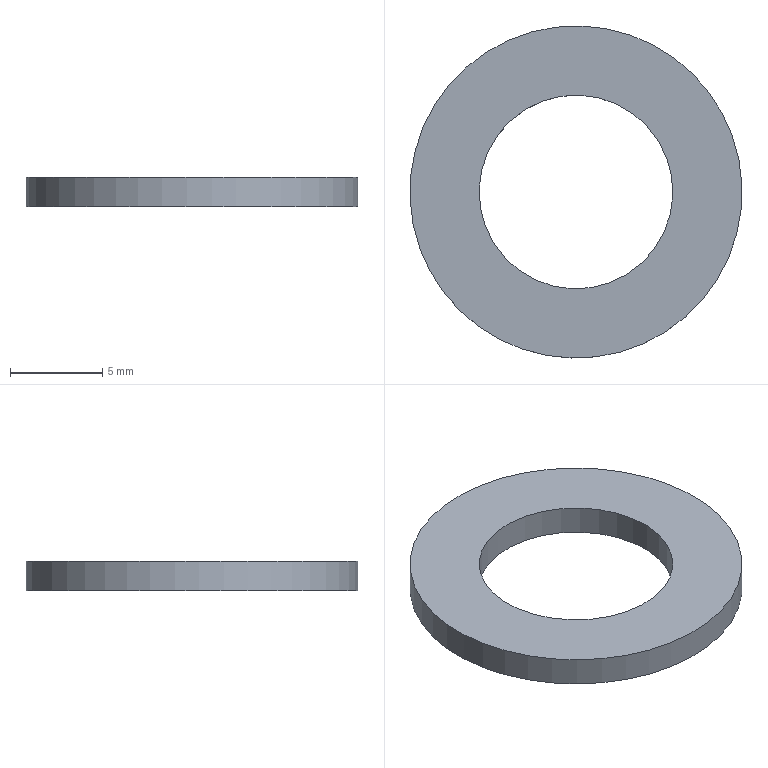Component | NX | CA6140-ZHUZHOU-DIANQUAN | 1 solid | 4 faces | box 18 x 18 x 1.6 mm | volume 269 mm3 | cylinder 2 | plane 2 | commonest cylinder face diameters 18 x1 10.5 x1
STEP:
#1=CARTESIAN_POINT('',(0.,0.,0.));
#2=DIRECTION('',(0.,0.,1.));
#3=DIRECTION('',(1.,0.,0.));
#4=AXIS2_PLACEMENT_3D('',#1,#2,#3);
#5=CARTESIAN_POINT('',(-61.859,-63.85,110.4));
#6=VERTEX_POINT('',#5);
#7=CARTESIAN_POINT('',(-56.569,-56.569,110.4));
#8=DIRECTION('',(0.,0.,1.));
#9=DIRECTION('',(-0.5878,-0.809,0.));
#10=AXIS2_PLACEMENT_3D('',#7,#8,#9);
#11=CIRCLE('',#10,9.);
#12=CARTESIAN_POINT('',(-56.569,-56.569,110.4));
#13=DIRECTION('',(0.,0.,1.));
#14=DIRECTION('',(0.5878,0.809,0.));
#15=AXIS2_PLACEMENT_3D('',#12,#13,#14);
#16=CYLINDRICAL_SURFACE('',#15,9.);
#17=CARTESIAN_POINT('',(3.142,0.));
#18=DIRECTION('',(1.,0.));
#19=VECTOR('',#18,1.);
#20=LINE('',#17,#19);
#21=(GEOMETRIC_REPRESENTATION_CONTEXT(2)PARAMETRIC_REPRESENTATION_CONTEXT()REPRESENTATION_CONTEXT('',''));
#22=DEFINITIONAL_REPRESENTATION('',(#20),#21);
#23=PCURVE('',#16,#22);
#24=CARTESIAN_POINT('',(-56.569,-56.569,110.4));
#25=DIRECTION('',(0.,0.,1.));
#26=DIRECTION('',(0.5878,0.809,0.));
#27=AXIS2_PLACEMENT_3D('',#24,#25,#26);
#28=PLANE('',#27);
#29=CARTESIAN_POINT('',(0.,0.));
#30=DIRECTION('',(-1.,0.));
#31=AXIS2_PLACEMENT_2D('',#29,#30);
#32=CIRCLE('',#31,9.);
#33=(GEOMETRIC_REPRESENTATION_CONTEXT(2)PARAMETRIC_REPRESENTATION_CONTEXT()REPRESENTATION_CONTEXT('',''));
#34=DEFINITIONAL_REPRESENTATION('',(#32),#33);
#35=PCURVE('',#28,#34);
#36=SURFACE_CURVE('',#11,(#23,#35),.PCURVE_S1.);
#37=EDGE_CURVE('',#6,#6,#36,.T.);
#38=ORIENTED_EDGE('',*,*,#37,.T.);
#39=CARTESIAN_POINT('',(-61.859,-63.85,112.));
#40=VERTEX_POINT('',#39);
#41=CARTESIAN_POINT('',(-61.859,-63.85,110.4));
#42=CARTESIAN_POINT('',(-61.859,-63.85,112.));
#43=B_SPLINE_CURVE_WITH_KNOTS('',1,(#41,#42),.UNSPECIFIED.,.F.,.F.,(2,2),(0.,1.6),.PIECEWISE_BEZIER_KNOTS.);
#44=CARTESIAN_POINT('',(9.425,0.));
#45=DIRECTION('',(0.,1.));
#46=VECTOR('',#45,1.);
#47=LINE('',#44,#46);
#48=(GEOMETRIC_REPRESENTATION_CONTEXT(2)PARAMETRIC_REPRESENTATION_CONTEXT()REPRESENTATION_CONTEXT('',''));
#49=DEFINITIONAL_REPRESENTATION('',(#47),#48);
#50=PCURVE('',#16,#49);
#51=CARTESIAN_POINT('',(3.142,0.));
#52=DIRECTION('',(0.,1.));
#53=VECTOR('',#52,1.);
#54=LINE('',#51,#53);
#55=(GEOMETRIC_REPRESENTATION_CONTEXT(2)PARAMETRIC_REPRESENTATION_CONTEXT()REPRESENTATION_CONTEXT('',''));
#56=DEFINITIONAL_REPRESENTATION('',(#54),#55);
#57=PCURVE('',#16,#56);
#58=SEAM_CURVE('',#43,(#50,#57),.PCURVE_S1.);
#59=EDGE_CURVE('',#6,#40,#58,.T.);
#60=ORIENTED_EDGE('',*,*,#59,.T.);
#61=CARTESIAN_POINT('',(-56.569,-56.569,112.));
#62=DIRECTION('',(0.,0.,1.));
#63=DIRECTION('',(-0.5878,-0.809,0.));
#64=AXIS2_PLACEMENT_3D('',#61,#62,#63);
#65=CIRCLE('',#64,9.);
#66=CARTESIAN_POINT('',(3.142,1.6));
#67=DIRECTION('',(1.,0.));
#68=VECTOR('',#67,1.);
#69=LINE('',#66,#68);
#70=(GEOMETRIC_REPRESENTATION_CONTEXT(2)PARAMETRIC_REPRESENTATION_CONTEXT()REPRESENTATION_CONTEXT('',''));
#71=DEFINITIONAL_REPRESENTATION('',(#69),#70);
#72=PCURVE('',#16,#71);
#73=CARTESIAN_POINT('',(-56.569,-56.569,112.));
#74=DIRECTION('',(0.,0.,1.));
#75=DIRECTION('',(0.5878,0.809,0.));
#76=AXIS2_PLACEMENT_3D('',#73,#74,#75);
#77=PLANE('',#76);
#78=CARTESIAN_POINT('',(0.,0.));
#79=DIRECTION('',(-1.,0.));
#80=AXIS2_PLACEMENT_2D('',#78,#79);
#81=CIRCLE('',#80,9.);
#82=(GEOMETRIC_REPRESENTATION_CONTEXT(2)PARAMETRIC_REPRESENTATION_CONTEXT()REPRESENTATION_CONTEXT('',''));
#83=DEFINITIONAL_REPRESENTATION('',(#81),#82);
#84=PCURVE('',#77,#83);
#85=SURFACE_CURVE('',#65,(#72,#84),.PCURVE_S1.);
#86=EDGE_CURVE('',#40,#40,#85,.T.);
#87=ORIENTED_EDGE('',*,*,#86,.F.);
#88=ORIENTED_EDGE('',*,*,#59,.F.);
#89=EDGE_LOOP('',(#38,#60,#87,#88));
#90=FACE_BOUND('',#89,.T.);
#91=ADVANCED_FACE('',(#90),#16,.T.);
#92=CARTESIAN_POINT('',(-59.654,-60.816,110.4));
#93=VERTEX_POINT('',#92);
#94=CARTESIAN_POINT('',(-56.569,-56.569,110.4));
#95=DIRECTION('',(0.,0.,1.));
#96=DIRECTION('',(-0.5878,-0.809,0.));
#97=AXIS2_PLACEMENT_3D('',#94,#95,#96);
#98=CIRCLE('',#97,5.25);
#99=CARTESIAN_POINT('',(-56.569,-56.569,110.4));
#100=DIRECTION('',(0.,0.,1.));
#101=DIRECTION('',(0.5878,0.809,0.));
#102=AXIS2_PLACEMENT_3D('',#99,#100,#101);
#103=CYLINDRICAL_SURFACE('',#102,5.25);
#104=CARTESIAN_POINT('',(3.142,0.));
#105=DIRECTION('',(1.,0.));
#106=VECTOR('',#105,1.);
#107=LINE('',#104,#106);
#108=(GEOMETRIC_REPRESENTATION_CONTEXT(2)PARAMETRIC_REPRESENTATION_CONTEXT()REPRESENTATION_CONTEXT('',''));
#109=DEFINITIONAL_REPRESENTATION('',(#107),#108);
#110=PCURVE('',#103,#109);
#111=CARTESIAN_POINT('',(0.,0.));
#112=DIRECTION('',(-1.,0.));
#113=AXIS2_PLACEMENT_2D('',#111,#112);
#114=CIRCLE('',#113,5.25);
#115=(GEOMETRIC_REPRESENTATION_CONTEXT(2)PARAMETRIC_REPRESENTATION_CONTEXT()REPRESENTATION_CONTEXT('',''));
#116=DEFINITIONAL_REPRESENTATION('',(#114),#115);
#117=PCURVE('',#28,#116);
#118=SURFACE_CURVE('',#98,(#110,#117),.PCURVE_S1.);
#119=EDGE_CURVE('',#93,#93,#118,.T.);
#120=ORIENTED_EDGE('',*,*,#119,.T.);
#121=CARTESIAN_POINT('',(-59.654,-60.816,112.));
#122=VERTEX_POINT('',#121);
#123=CARTESIAN_POINT('',(-59.654,-60.816,110.4));
#124=CARTESIAN_POINT('',(-59.654,-60.816,112.));
#125=B_SPLINE_CURVE_WITH_KNOTS('',1,(#123,#124),.UNSPECIFIED.,.F.,.F.,(2,2),(0.,1.6),.PIECEWISE_BEZIER_KNOTS.);
#126=CARTESIAN_POINT('',(9.425,0.));
#127=DIRECTION('',(0.,1.));
#128=VECTOR('',#127,1.);
#129=LINE('',#126,#128);
#130=(GEOMETRIC_REPRESENTATION_CONTEXT(2)PARAMETRIC_REPRESENTATION_CONTEXT()REPRESENTATION_CONTEXT('',''));
#131=DEFINITIONAL_REPRESENTATION('',(#129),#130);
#132=PCURVE('',#103,#131);
#133=CARTESIAN_POINT('',(3.142,0.));
#134=DIRECTION('',(0.,1.));
#135=VECTOR('',#134,1.);
#136=LINE('',#133,#135);
#137=(GEOMETRIC_REPRESENTATION_CONTEXT(2)PARAMETRIC_REPRESENTATION_CONTEXT()REPRESENTATION_CONTEXT('',''));
#138=DEFINITIONAL_REPRESENTATION('',(#136),#137);
#139=PCURVE('',#103,#138);
#140=SEAM_CURVE('',#125,(#132,#139),.PCURVE_S1.);
#141=EDGE_CURVE('',#93,#122,#140,.T.);
#142=ORIENTED_EDGE('',*,*,#141,.T.);
#143=CARTESIAN_POINT('',(-56.569,-56.569,112.));
#144=DIRECTION('',(0.,0.,1.));
#145=DIRECTION('',(-0.5878,-0.809,0.));
#146=AXIS2_PLACEMENT_3D('',#143,#144,#145);
#147=CIRCLE('',#146,5.25);
#148=CARTESIAN_POINT('',(3.142,1.6));
#149=DIRECTION('',(1.,0.));
#150=VECTOR('',#149,1.);
#151=LINE('',#148,#150);
#152=(GEOMETRIC_REPRESENTATION_CONTEXT(2)PARAMETRIC_REPRESENTATION_CONTEXT()REPRESENTATION_CONTEXT('',''));
#153=DEFINITIONAL_REPRESENTATION('',(#151),#152);
#154=PCURVE('',#103,#153);
#155=CARTESIAN_POINT('',(0.,0.));
#156=DIRECTION('',(-1.,0.));
#157=AXIS2_PLACEMENT_2D('',#155,#156);
#158=CIRCLE('',#157,5.25);
#159=(GEOMETRIC_REPRESENTATION_CONTEXT(2)PARAMETRIC_REPRESENTATION_CONTEXT()REPRESENTATION_CONTEXT('',''));
#160=DEFINITIONAL_REPRESENTATION('',(#158),#159);
#161=PCURVE('',#77,#160);
#162=SURFACE_CURVE('',#147,(#154,#161),.PCURVE_S1.);
#163=EDGE_CURVE('',#122,#122,#162,.T.);
#164=ORIENTED_EDGE('',*,*,#163,.F.);
#165=ORIENTED_EDGE('',*,*,#141,.F.);
#166=EDGE_LOOP('',(#120,#142,#164,#165));
#167=FACE_BOUND('',#166,.F.);
#168=ADVANCED_FACE('',(#167),#103,.F.);
#169=ORIENTED_EDGE('',*,*,#37,.F.);
#170=EDGE_LOOP('',(#169));
#171=FACE_BOUND('',#170,.T.);
#172=ORIENTED_EDGE('',*,*,#119,.T.);
#173=EDGE_LOOP('',(#172));
#174=FACE_BOUND('',#173,.T.);
#175=ADVANCED_FACE('',(#171,#174),#28,.F.);
#176=ORIENTED_EDGE('',*,*,#86,.T.);
#177=EDGE_LOOP('',(#176));
#178=FACE_BOUND('',#177,.T.);
#179=ORIENTED_EDGE('',*,*,#163,.F.);
#180=EDGE_LOOP('',(#179));
#181=FACE_BOUND('',#180,.T.);
#182=ADVANCED_FACE('',(#178,#181),#77,.T.);
#183=CLOSED_SHELL('',(#91,#168,#175,#182));
#184=MANIFOLD_SOLID_BREP('',#183);
#185=(LENGTH_UNIT()NAMED_UNIT(*)SI_UNIT(.MILLI.,.METRE.));
#186=UNCERTAINTY_MEASURE_WITH_UNIT(LENGTH_MEASURE(0.00001),#185,'','');
#187=(NAMED_UNIT(*)PLANE_ANGLE_UNIT()SI_UNIT($,.RADIAN.));
#188=(NAMED_UNIT(*)SI_UNIT($,.STERADIAN.)SOLID_ANGLE_UNIT());
#189=(GEOMETRIC_REPRESENTATION_CONTEXT(3)GLOBAL_UNCERTAINTY_ASSIGNED_CONTEXT((#186))GLOBAL_UNIT_ASSIGNED_CONTEXT((#185,#187,#188))REPRESENTATION_CONTEXT('',''));
#190=ADVANCED_BREP_SHAPE_REPRESENTATION('',(#4,#184),#189);